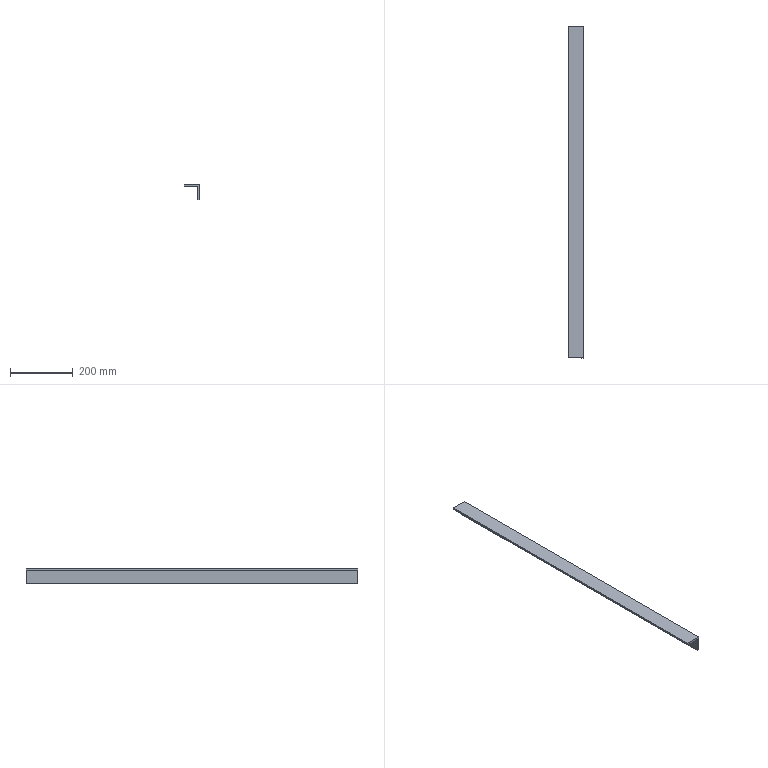Component | NX | WIDTH_CORNER_PROTECTOR | 1 solid | 8 faces | box 50 x 1054 x 50 mm | volume 594456 mm3 | plane 8
STEP:
#1=CARTESIAN_POINT('',(0.,0.,0.));
#2=DIRECTION('',(0.,0.,1.));
#3=DIRECTION('',(1.,0.,0.));
#4=AXIS2_PLACEMENT_3D('',#1,#2,#3);
#5=CARTESIAN_POINT('',(639.5,-527.,937.));
#6=VERTEX_POINT('',#5);
#7=CARTESIAN_POINT('',(639.5,-527.,987.));
#8=VERTEX_POINT('',#7);
#9=CARTESIAN_POINT('',(639.5,-527.,981.));
#10=DIRECTION('',(0.,0.,1.));
#11=VECTOR('',#10,1.);
#12=LINE('',#9,#11);
#13=CARTESIAN_POINT('',(628.5,-527.,0.));
#14=DIRECTION('',(-0.,-1.,0.));
#15=DIRECTION('',(1.,-0.,-0.));
#16=AXIS2_PLACEMENT_3D('',#13,#14,#15);
#17=PLANE('',#16);
#18=CARTESIAN_POINT('',(11.,981.));
#19=DIRECTION('',(-0.,1.));
#20=VECTOR('',#19,1.);
#21=LINE('',#18,#20);
#22=(GEOMETRIC_REPRESENTATION_CONTEXT(2)PARAMETRIC_REPRESENTATION_CONTEXT()REPRESENTATION_CONTEXT('',''));
#23=DEFINITIONAL_REPRESENTATION('',(#21),#22);
#24=PCURVE('',#17,#23);
#25=CARTESIAN_POINT('',(639.5,527.,981.));
#26=DIRECTION('',(-1.,0.,0.));
#27=DIRECTION('',(0.,0.,-1.));
#28=AXIS2_PLACEMENT_3D('',#25,#26,#27);
#29=PLANE('',#28);
#30=CARTESIAN_POINT('',(0.,1054.));
#31=DIRECTION('',(-1.,-0.));
#32=VECTOR('',#31,1.);
#33=LINE('',#30,#32);
#34=(GEOMETRIC_REPRESENTATION_CONTEXT(2)PARAMETRIC_REPRESENTATION_CONTEXT()REPRESENTATION_CONTEXT('',''));
#35=DEFINITIONAL_REPRESENTATION('',(#33),#34);
#36=PCURVE('',#29,#35);
#37=SURFACE_CURVE('',#12,(#24,#36),.PCURVE_S1.);
#38=EDGE_CURVE('',#6,#8,#37,.T.);
#39=ORIENTED_EDGE('',*,*,#38,.T.);
#40=CARTESIAN_POINT('',(589.5,-527.,987.));
#41=VERTEX_POINT('',#40);
#42=CARTESIAN_POINT('',(-628.5,-527.,987.));
#43=DIRECTION('',(-1.,0.,0.));
#44=VECTOR('',#43,1.);
#45=LINE('',#42,#44);
#46=CARTESIAN_POINT('',(-1257.,987.));
#47=DIRECTION('',(-1.,-0.));
#48=VECTOR('',#47,1.);
#49=LINE('',#46,#48);
#50=(GEOMETRIC_REPRESENTATION_CONTEXT(2)PARAMETRIC_REPRESENTATION_CONTEXT()REPRESENTATION_CONTEXT('',''));
#51=DEFINITIONAL_REPRESENTATION('',(#49),#50);
#52=PCURVE('',#17,#51);
#53=CARTESIAN_POINT('',(-628.5,527.,987.));
#54=DIRECTION('',(0.,0.,-1.));
#55=DIRECTION('',(1.,0.,0.));
#56=AXIS2_PLACEMENT_3D('',#53,#54,#55);
#57=PLANE('',#56);
#58=CARTESIAN_POINT('',(0.,1054.));
#59=DIRECTION('',(-1.,-0.));
#60=VECTOR('',#59,1.);
#61=LINE('',#58,#60);
#62=(GEOMETRIC_REPRESENTATION_CONTEXT(2)PARAMETRIC_REPRESENTATION_CONTEXT()REPRESENTATION_CONTEXT('',''));
#63=DEFINITIONAL_REPRESENTATION('',(#61),#62);
#64=PCURVE('',#57,#63);
#65=SURFACE_CURVE('',#45,(#52,#64),.PCURVE_S1.);
#66=EDGE_CURVE('',#8,#41,#65,.T.);
#67=ORIENTED_EDGE('',*,*,#66,.T.);
#68=CARTESIAN_POINT('',(589.5,-527.,981.));
#69=VERTEX_POINT('',#68);
#70=CARTESIAN_POINT('',(589.5,-527.,981.));
#71=DIRECTION('',(0.,-0.,-1.));
#72=VECTOR('',#71,1.);
#73=LINE('',#70,#72);
#74=CARTESIAN_POINT('',(-39.,981.));
#75=DIRECTION('',(0.,-1.));
#76=VECTOR('',#75,1.);
#77=LINE('',#74,#76);
#78=(GEOMETRIC_REPRESENTATION_CONTEXT(2)PARAMETRIC_REPRESENTATION_CONTEXT()REPRESENTATION_CONTEXT('',''));
#79=DEFINITIONAL_REPRESENTATION('',(#77),#78);
#80=PCURVE('',#17,#79);
#81=CARTESIAN_POINT('',(589.5,527.,981.));
#82=DIRECTION('',(1.,0.,0.));
#83=DIRECTION('',(0.,-1.,0.));
#84=AXIS2_PLACEMENT_3D('',#81,#82,#83);
#85=PLANE('',#84);
#86=CARTESIAN_POINT('',(1054.,0.));
#87=DIRECTION('',(0.,1.));
#88=VECTOR('',#87,1.);
#89=LINE('',#86,#88);
#90=(GEOMETRIC_REPRESENTATION_CONTEXT(2)PARAMETRIC_REPRESENTATION_CONTEXT()REPRESENTATION_CONTEXT('',''));
#91=DEFINITIONAL_REPRESENTATION('',(#89),#90);
#92=PCURVE('',#85,#91);
#93=SURFACE_CURVE('',#73,(#80,#92),.PCURVE_S1.);
#94=EDGE_CURVE('',#41,#69,#93,.T.);
#95=ORIENTED_EDGE('',*,*,#94,.T.);
#96=CARTESIAN_POINT('',(633.5,-527.,981.));
#97=VERTEX_POINT('',#96);
#98=CARTESIAN_POINT('',(-628.5,-527.,981.));
#99=DIRECTION('',(-1.,0.,0.));
#100=VECTOR('',#99,1.);
#101=LINE('',#98,#100);
#102=CARTESIAN_POINT('',(-1257.,981.));
#103=DIRECTION('',(-1.,-0.));
#104=VECTOR('',#103,1.);
#105=LINE('',#102,#104);
#106=(GEOMETRIC_REPRESENTATION_CONTEXT(2)PARAMETRIC_REPRESENTATION_CONTEXT()REPRESENTATION_CONTEXT('',''));
#107=DEFINITIONAL_REPRESENTATION('',(#105),#106);
#108=PCURVE('',#17,#107);
#109=CARTESIAN_POINT('',(-628.5,527.,981.));
#110=DIRECTION('',(0.,0.,-1.));
#111=DIRECTION('',(1.,0.,0.));
#112=AXIS2_PLACEMENT_3D('',#109,#110,#111);
#113=PLANE('',#112);
#114=CARTESIAN_POINT('',(0.,1054.));
#115=DIRECTION('',(-1.,-0.));
#116=VECTOR('',#115,1.);
#117=LINE('',#114,#116);
#118=(GEOMETRIC_REPRESENTATION_CONTEXT(2)PARAMETRIC_REPRESENTATION_CONTEXT()REPRESENTATION_CONTEXT('',''));
#119=DEFINITIONAL_REPRESENTATION('',(#117),#118);
#120=PCURVE('',#113,#119);
#121=SURFACE_CURVE('',#101,(#108,#120),.PCURVE_S1.);
#122=EDGE_CURVE('',#97,#69,#121,.T.);
#123=ORIENTED_EDGE('',*,*,#122,.F.);
#124=CARTESIAN_POINT('',(633.5,-527.,937.));
#125=VERTEX_POINT('',#124);
#126=CARTESIAN_POINT('',(633.5,-527.,981.));
#127=DIRECTION('',(0.,0.,1.));
#128=VECTOR('',#127,1.);
#129=LINE('',#126,#128);
#130=CARTESIAN_POINT('',(5.,981.));
#131=DIRECTION('',(-0.,1.));
#132=VECTOR('',#131,1.);
#133=LINE('',#130,#132);
#134=(GEOMETRIC_REPRESENTATION_CONTEXT(2)PARAMETRIC_REPRESENTATION_CONTEXT()REPRESENTATION_CONTEXT('',''));
#135=DEFINITIONAL_REPRESENTATION('',(#133),#134);
#136=PCURVE('',#17,#135);
#137=CARTESIAN_POINT('',(633.5,527.,981.));
#138=DIRECTION('',(-1.,0.,0.));
#139=DIRECTION('',(0.,0.,-1.));
#140=AXIS2_PLACEMENT_3D('',#137,#138,#139);
#141=PLANE('',#140);
#142=CARTESIAN_POINT('',(0.,1054.));
#143=DIRECTION('',(-1.,-0.));
#144=VECTOR('',#143,1.);
#145=LINE('',#142,#144);
#146=(GEOMETRIC_REPRESENTATION_CONTEXT(2)PARAMETRIC_REPRESENTATION_CONTEXT()REPRESENTATION_CONTEXT('',''));
#147=DEFINITIONAL_REPRESENTATION('',(#145),#146);
#148=PCURVE('',#141,#147);
#149=SURFACE_CURVE('',#129,(#136,#148),.PCURVE_S1.);
#150=EDGE_CURVE('',#125,#97,#149,.T.);
#151=ORIENTED_EDGE('',*,*,#150,.F.);
#152=CARTESIAN_POINT('',(633.5,-527.,937.));
#153=DIRECTION('',(1.,-0.,0.));
#154=VECTOR('',#153,1.);
#155=LINE('',#152,#154);
#156=CARTESIAN_POINT('',(5.,937.));
#157=DIRECTION('',(1.,0.));
#158=VECTOR('',#157,1.);
#159=LINE('',#156,#158);
#160=(GEOMETRIC_REPRESENTATION_CONTEXT(2)PARAMETRIC_REPRESENTATION_CONTEXT()REPRESENTATION_CONTEXT('',''));
#161=DEFINITIONAL_REPRESENTATION('',(#159),#160);
#162=PCURVE('',#17,#161);
#163=CARTESIAN_POINT('',(633.5,527.,937.));
#164=DIRECTION('',(0.,0.,-1.));
#165=DIRECTION('',(0.,-1.,0.));
#166=AXIS2_PLACEMENT_3D('',#163,#164,#165);
#167=PLANE('',#166);
#168=CARTESIAN_POINT('',(1054.,0.));
#169=DIRECTION('',(0.,-1.));
#170=VECTOR('',#169,1.);
#171=LINE('',#168,#170);
#172=(GEOMETRIC_REPRESENTATION_CONTEXT(2)PARAMETRIC_REPRESENTATION_CONTEXT()REPRESENTATION_CONTEXT('',''));
#173=DEFINITIONAL_REPRESENTATION('',(#171),#172);
#174=PCURVE('',#167,#173);
#175=SURFACE_CURVE('',#155,(#162,#174),.PCURVE_S1.);
#176=EDGE_CURVE('',#125,#6,#175,.T.);
#177=ORIENTED_EDGE('',*,*,#176,.T.);
#178=EDGE_LOOP('',(#39,#67,#95,#123,#151,#177));
#179=FACE_BOUND('',#178,.T.);
#180=ADVANCED_FACE('',(#179),#17,.T.);
#181=ORIENTED_EDGE('',*,*,#66,.F.);
#182=CARTESIAN_POINT('',(639.5,527.,987.));
#183=VERTEX_POINT('',#182);
#184=CARTESIAN_POINT('',(639.5,527.,987.));
#185=DIRECTION('',(0.,-1.,0.));
#186=VECTOR('',#185,1.);
#187=LINE('',#184,#186);
#188=CARTESIAN_POINT('',(1268.,0.));
#189=DIRECTION('',(0.,1.));
#190=VECTOR('',#189,1.);
#191=LINE('',#188,#190);
#192=(GEOMETRIC_REPRESENTATION_CONTEXT(2)PARAMETRIC_REPRESENTATION_CONTEXT()REPRESENTATION_CONTEXT('',''));
#193=DEFINITIONAL_REPRESENTATION('',(#191),#192);
#194=PCURVE('',#57,#193);
#195=CARTESIAN_POINT('',(-6.,0.));
#196=DIRECTION('',(0.,1.));
#197=VECTOR('',#196,1.);
#198=LINE('',#195,#197);
#199=(GEOMETRIC_REPRESENTATION_CONTEXT(2)PARAMETRIC_REPRESENTATION_CONTEXT()REPRESENTATION_CONTEXT('',''));
#200=DEFINITIONAL_REPRESENTATION('',(#198),#199);
#201=PCURVE('',#29,#200);
#202=SURFACE_CURVE('',#187,(#194,#201),.PCURVE_S1.);
#203=EDGE_CURVE('',#183,#8,#202,.T.);
#204=ORIENTED_EDGE('',*,*,#203,.F.);
#205=CARTESIAN_POINT('',(589.5,527.,987.));
#206=VERTEX_POINT('',#205);
#207=CARTESIAN_POINT('',(-628.5,527.,987.));
#208=DIRECTION('',(1.,0.,0.));
#209=VECTOR('',#208,1.);
#210=LINE('',#207,#209);
#211=CARTESIAN_POINT('',(0.,0.));
#212=DIRECTION('',(1.,0.));
#213=VECTOR('',#212,1.);
#214=LINE('',#211,#213);
#215=(GEOMETRIC_REPRESENTATION_CONTEXT(2)PARAMETRIC_REPRESENTATION_CONTEXT()REPRESENTATION_CONTEXT('',''));
#216=DEFINITIONAL_REPRESENTATION('',(#214),#215);
#217=PCURVE('',#57,#216);
#218=CARTESIAN_POINT('',(633.5,527.,981.));
#219=DIRECTION('',(0.,1.,0.));
#220=DIRECTION('',(0.,0.,-1.));
#221=AXIS2_PLACEMENT_3D('',#218,#219,#220);
#222=PLANE('',#221);
#223=CARTESIAN_POINT('',(-6.,1262.));
#224=DIRECTION('',(0.,-1.));
#225=VECTOR('',#224,1.);
#226=LINE('',#223,#225);
#227=(GEOMETRIC_REPRESENTATION_CONTEXT(2)PARAMETRIC_REPRESENTATION_CONTEXT()REPRESENTATION_CONTEXT('',''));
#228=DEFINITIONAL_REPRESENTATION('',(#226),#227);
#229=PCURVE('',#222,#228);
#230=SURFACE_CURVE('',#210,(#217,#229),.PCURVE_S1.);
#231=EDGE_CURVE('',#206,#183,#230,.T.);
#232=ORIENTED_EDGE('',*,*,#231,.F.);
#233=CARTESIAN_POINT('',(589.5,527.,987.));
#234=DIRECTION('',(0.,-1.,0.));
#235=VECTOR('',#234,1.);
#236=LINE('',#233,#235);
#237=CARTESIAN_POINT('',(1218.,0.));
#238=DIRECTION('',(0.,1.));
#239=VECTOR('',#238,1.);
#240=LINE('',#237,#239);
#241=(GEOMETRIC_REPRESENTATION_CONTEXT(2)PARAMETRIC_REPRESENTATION_CONTEXT()REPRESENTATION_CONTEXT('',''));
#242=DEFINITIONAL_REPRESENTATION('',(#240),#241);
#243=PCURVE('',#57,#242);
#244=CARTESIAN_POINT('',(0.,-6.));
#245=DIRECTION('',(1.,0.));
#246=VECTOR('',#245,1.);
#247=LINE('',#244,#246);
#248=(GEOMETRIC_REPRESENTATION_CONTEXT(2)PARAMETRIC_REPRESENTATION_CONTEXT()REPRESENTATION_CONTEXT('',''));
#249=DEFINITIONAL_REPRESENTATION('',(#247),#248);
#250=PCURVE('',#85,#249);
#251=SURFACE_CURVE('',#236,(#243,#250),.PCURVE_S1.);
#252=EDGE_CURVE('',#206,#41,#251,.T.);
#253=ORIENTED_EDGE('',*,*,#252,.T.);
#254=EDGE_LOOP('',(#181,#204,#232,#253));
#255=FACE_BOUND('',#254,.T.);
#256=ADVANCED_FACE('',(#255),#57,.F.);
#257=ORIENTED_EDGE('',*,*,#94,.F.);
#258=ORIENTED_EDGE('',*,*,#252,.F.);
#259=CARTESIAN_POINT('',(589.5,527.,981.));
#260=VERTEX_POINT('',#259);
#261=CARTESIAN_POINT('',(589.5,527.,981.));
#262=DIRECTION('',(0.,0.,1.));
#263=VECTOR('',#262,1.);
#264=LINE('',#261,#263);
#265=CARTESIAN_POINT('',(0.,0.));
#266=DIRECTION('',(0.,-1.));
#267=VECTOR('',#266,1.);
#268=LINE('',#265,#267);
#269=(GEOMETRIC_REPRESENTATION_CONTEXT(2)PARAMETRIC_REPRESENTATION_CONTEXT()REPRESENTATION_CONTEXT('',''));
#270=DEFINITIONAL_REPRESENTATION('',(#268),#269);
#271=PCURVE('',#85,#270);
#272=CARTESIAN_POINT('',(0.,44.));
#273=DIRECTION('',(-1.,0.));
#274=VECTOR('',#273,1.);
#275=LINE('',#272,#274);
#276=(GEOMETRIC_REPRESENTATION_CONTEXT(2)PARAMETRIC_REPRESENTATION_CONTEXT()REPRESENTATION_CONTEXT('',''));
#277=DEFINITIONAL_REPRESENTATION('',(#275),#276);
#278=PCURVE('',#222,#277);
#279=SURFACE_CURVE('',#264,(#271,#278),.PCURVE_S1.);
#280=EDGE_CURVE('',#260,#206,#279,.T.);
#281=ORIENTED_EDGE('',*,*,#280,.F.);
#282=CARTESIAN_POINT('',(589.5,527.,981.));
#283=DIRECTION('',(0.,-1.,0.));
#284=VECTOR('',#283,1.);
#285=LINE('',#282,#284);
#286=CARTESIAN_POINT('',(0.,0.));
#287=DIRECTION('',(1.,0.));
#288=VECTOR('',#287,1.);
#289=LINE('',#286,#288);
#290=(GEOMETRIC_REPRESENTATION_CONTEXT(2)PARAMETRIC_REPRESENTATION_CONTEXT()REPRESENTATION_CONTEXT('',''));
#291=DEFINITIONAL_REPRESENTATION('',(#289),#290);
#292=PCURVE('',#85,#291);
#293=CARTESIAN_POINT('',(1218.,0.));
#294=DIRECTION('',(0.,1.));
#295=VECTOR('',#294,1.);
#296=LINE('',#293,#295);
#297=(GEOMETRIC_REPRESENTATION_CONTEXT(2)PARAMETRIC_REPRESENTATION_CONTEXT()REPRESENTATION_CONTEXT('',''));
#298=DEFINITIONAL_REPRESENTATION('',(#296),#297);
#299=PCURVE('',#113,#298);
#300=SURFACE_CURVE('',#285,(#292,#299),.PCURVE_S1.);
#301=EDGE_CURVE('',#260,#69,#300,.T.);
#302=ORIENTED_EDGE('',*,*,#301,.T.);
#303=EDGE_LOOP('',(#257,#258,#281,#302));
#304=FACE_BOUND('',#303,.T.);
#305=ADVANCED_FACE('',(#304),#85,.F.);
#306=CARTESIAN_POINT('',(633.5,527.,981.));
#307=VERTEX_POINT('',#306);
#308=CARTESIAN_POINT('',(633.5,527.,937.));
#309=VERTEX_POINT('',#308);
#310=CARTESIAN_POINT('',(633.5,527.,981.));
#311=DIRECTION('',(0.,0.,-1.));
#312=VECTOR('',#311,1.);
#313=LINE('',#310,#312);
#314=CARTESIAN_POINT('',(0.,0.));
#315=DIRECTION('',(1.,0.));
#316=VECTOR('',#315,1.);
#317=LINE('',#314,#316);
#318=(GEOMETRIC_REPRESENTATION_CONTEXT(2)PARAMETRIC_REPRESENTATION_CONTEXT()REPRESENTATION_CONTEXT('',''));
#319=DEFINITIONAL_REPRESENTATION('',(#317),#318);
#320=PCURVE('',#222,#319);
#321=CARTESIAN_POINT('',(0.,0.));
#322=DIRECTION('',(1.,0.));
#323=VECTOR('',#322,1.);
#324=LINE('',#321,#323);
#325=(GEOMETRIC_REPRESENTATION_CONTEXT(2)PARAMETRIC_REPRESENTATION_CONTEXT()REPRESENTATION_CONTEXT('',''));
#326=DEFINITIONAL_REPRESENTATION('',(#324),#325);
#327=PCURVE('',#141,#326);
#328=SURFACE_CURVE('',#313,(#320,#327),.PCURVE_S1.);
#329=EDGE_CURVE('',#307,#309,#328,.T.);
#330=ORIENTED_EDGE('',*,*,#329,.F.);
#331=CARTESIAN_POINT('',(-628.5,527.,981.));
#332=DIRECTION('',(1.,-0.,0.));
#333=VECTOR('',#332,1.);
#334=LINE('',#331,#333);
#335=CARTESIAN_POINT('',(0.,1262.));
#336=DIRECTION('',(0.,-1.));
#337=VECTOR('',#336,1.);
#338=LINE('',#335,#337);
#339=(GEOMETRIC_REPRESENTATION_CONTEXT(2)PARAMETRIC_REPRESENTATION_CONTEXT()REPRESENTATION_CONTEXT('',''));
#340=DEFINITIONAL_REPRESENTATION('',(#338),#339);
#341=PCURVE('',#222,#340);
#342=CARTESIAN_POINT('',(0.,0.));
#343=DIRECTION('',(1.,0.));
#344=VECTOR('',#343,1.);
#345=LINE('',#342,#344);
#346=(GEOMETRIC_REPRESENTATION_CONTEXT(2)PARAMETRIC_REPRESENTATION_CONTEXT()REPRESENTATION_CONTEXT('',''));
#347=DEFINITIONAL_REPRESENTATION('',(#345),#346);
#348=PCURVE('',#113,#347);
#349=SURFACE_CURVE('',#334,(#341,#348),.PCURVE_S1.);
#350=EDGE_CURVE('',#260,#307,#349,.T.);
#351=ORIENTED_EDGE('',*,*,#350,.F.);
#352=ORIENTED_EDGE('',*,*,#280,.T.);
#353=ORIENTED_EDGE('',*,*,#231,.T.);
#354=CARTESIAN_POINT('',(639.5,527.,937.));
#355=VERTEX_POINT('',#354);
#356=CARTESIAN_POINT('',(639.5,527.,981.));
#357=DIRECTION('',(0.,0.,-1.));
#358=VECTOR('',#357,1.);
#359=LINE('',#356,#358);
#360=CARTESIAN_POINT('',(0.,-6.));
#361=DIRECTION('',(1.,0.));
#362=VECTOR('',#361,1.);
#363=LINE('',#360,#362);
#364=(GEOMETRIC_REPRESENTATION_CONTEXT(2)PARAMETRIC_REPRESENTATION_CONTEXT()REPRESENTATION_CONTEXT('',''));
#365=DEFINITIONAL_REPRESENTATION('',(#363),#364);
#366=PCURVE('',#222,#365);
#367=CARTESIAN_POINT('',(0.,0.));
#368=DIRECTION('',(1.,0.));
#369=VECTOR('',#368,1.);
#370=LINE('',#367,#369);
#371=(GEOMETRIC_REPRESENTATION_CONTEXT(2)PARAMETRIC_REPRESENTATION_CONTEXT()REPRESENTATION_CONTEXT('',''));
#372=DEFINITIONAL_REPRESENTATION('',(#370),#371);
#373=PCURVE('',#29,#372);
#374=SURFACE_CURVE('',#359,(#366,#373),.PCURVE_S1.);
#375=EDGE_CURVE('',#183,#355,#374,.T.);
#376=ORIENTED_EDGE('',*,*,#375,.T.);
#377=CARTESIAN_POINT('',(633.5,527.,937.));
#378=DIRECTION('',(1.,0.,0.));
#379=VECTOR('',#378,1.);
#380=LINE('',#377,#379);
#381=CARTESIAN_POINT('',(44.,0.));
#382=DIRECTION('',(0.,-1.));
#383=VECTOR('',#382,1.);
#384=LINE('',#381,#383);
#385=(GEOMETRIC_REPRESENTATION_CONTEXT(2)PARAMETRIC_REPRESENTATION_CONTEXT()REPRESENTATION_CONTEXT('',''));
#386=DEFINITIONAL_REPRESENTATION('',(#384),#385);
#387=PCURVE('',#222,#386);
#388=CARTESIAN_POINT('',(0.,0.));
#389=DIRECTION('',(0.,-1.));
#390=VECTOR('',#389,1.);
#391=LINE('',#388,#390);
#392=(GEOMETRIC_REPRESENTATION_CONTEXT(2)PARAMETRIC_REPRESENTATION_CONTEXT()REPRESENTATION_CONTEXT('',''));
#393=DEFINITIONAL_REPRESENTATION('',(#391),#392);
#394=PCURVE('',#167,#393);
#395=SURFACE_CURVE('',#380,(#387,#394),.PCURVE_S1.);
#396=EDGE_CURVE('',#309,#355,#395,.T.);
#397=ORIENTED_EDGE('',*,*,#396,.F.);
#398=EDGE_LOOP('',(#330,#351,#352,#353,#376,#397));
#399=FACE_BOUND('',#398,.T.);
#400=ADVANCED_FACE('',(#399),#222,.T.);
#401=CARTESIAN_POINT('',(633.5,527.,981.));
#402=DIRECTION('',(0.,-1.,0.));
#403=VECTOR('',#402,1.);
#404=LINE('',#401,#403);
#405=CARTESIAN_POINT('',(1262.,0.));
#406=DIRECTION('',(0.,1.));
#407=VECTOR('',#406,1.);
#408=LINE('',#405,#407);
#409=(GEOMETRIC_REPRESENTATION_CONTEXT(2)PARAMETRIC_REPRESENTATION_CONTEXT()REPRESENTATION_CONTEXT('',''));
#410=DEFINITIONAL_REPRESENTATION('',(#408),#409);
#411=PCURVE('',#113,#410);
#412=CARTESIAN_POINT('',(0.,0.));
#413=DIRECTION('',(0.,1.));
#414=VECTOR('',#413,1.);
#415=LINE('',#412,#414);
#416=(GEOMETRIC_REPRESENTATION_CONTEXT(2)PARAMETRIC_REPRESENTATION_CONTEXT()REPRESENTATION_CONTEXT('',''));
#417=DEFINITIONAL_REPRESENTATION('',(#415),#416);
#418=PCURVE('',#141,#417);
#419=SURFACE_CURVE('',#404,(#411,#418),.PCURVE_S1.);
#420=EDGE_CURVE('',#307,#97,#419,.T.);
#421=ORIENTED_EDGE('',*,*,#420,.T.);
#422=ORIENTED_EDGE('',*,*,#122,.T.);
#423=ORIENTED_EDGE('',*,*,#301,.F.);
#424=ORIENTED_EDGE('',*,*,#350,.T.);
#425=EDGE_LOOP('',(#421,#422,#423,#424));
#426=FACE_BOUND('',#425,.T.);
#427=ADVANCED_FACE('',(#426),#113,.T.);
#428=ORIENTED_EDGE('',*,*,#176,.F.);
#429=CARTESIAN_POINT('',(633.5,527.,937.));
#430=DIRECTION('',(0.,-1.,0.));
#431=VECTOR('',#430,1.);
#432=LINE('',#429,#431);
#433=CARTESIAN_POINT('',(0.,0.));
#434=DIRECTION('',(1.,0.));
#435=VECTOR('',#434,1.);
#436=LINE('',#433,#435);
#437=(GEOMETRIC_REPRESENTATION_CONTEXT(2)PARAMETRIC_REPRESENTATION_CONTEXT()REPRESENTATION_CONTEXT('',''));
#438=DEFINITIONAL_REPRESENTATION('',(#436),#437);
#439=PCURVE('',#167,#438);
#440=CARTESIAN_POINT('',(44.,0.));
#441=DIRECTION('',(0.,1.));
#442=VECTOR('',#441,1.);
#443=LINE('',#440,#442);
#444=(GEOMETRIC_REPRESENTATION_CONTEXT(2)PARAMETRIC_REPRESENTATION_CONTEXT()REPRESENTATION_CONTEXT('',''));
#445=DEFINITIONAL_REPRESENTATION('',(#443),#444);
#446=PCURVE('',#141,#445);
#447=SURFACE_CURVE('',#432,(#439,#446),.PCURVE_S1.);
#448=EDGE_CURVE('',#309,#125,#447,.T.);
#449=ORIENTED_EDGE('',*,*,#448,.F.);
#450=ORIENTED_EDGE('',*,*,#396,.T.);
#451=CARTESIAN_POINT('',(639.5,527.,937.));
#452=DIRECTION('',(0.,-1.,0.));
#453=VECTOR('',#452,1.);
#454=LINE('',#451,#453);
#455=CARTESIAN_POINT('',(0.,-6.));
#456=DIRECTION('',(1.,0.));
#457=VECTOR('',#456,1.);
#458=LINE('',#455,#457);
#459=(GEOMETRIC_REPRESENTATION_CONTEXT(2)PARAMETRIC_REPRESENTATION_CONTEXT()REPRESENTATION_CONTEXT('',''));
#460=DEFINITIONAL_REPRESENTATION('',(#458),#459);
#461=PCURVE('',#167,#460);
#462=CARTESIAN_POINT('',(44.,0.));
#463=DIRECTION('',(0.,1.));
#464=VECTOR('',#463,1.);
#465=LINE('',#462,#464);
#466=(GEOMETRIC_REPRESENTATION_CONTEXT(2)PARAMETRIC_REPRESENTATION_CONTEXT()REPRESENTATION_CONTEXT('',''));
#467=DEFINITIONAL_REPRESENTATION('',(#465),#466);
#468=PCURVE('',#29,#467);
#469=SURFACE_CURVE('',#454,(#461,#468),.PCURVE_S1.);
#470=EDGE_CURVE('',#355,#6,#469,.T.);
#471=ORIENTED_EDGE('',*,*,#470,.T.);
#472=EDGE_LOOP('',(#428,#449,#450,#471));
#473=FACE_BOUND('',#472,.T.);
#474=ADVANCED_FACE('',(#473),#167,.T.);
#475=ORIENTED_EDGE('',*,*,#448,.T.);
#476=ORIENTED_EDGE('',*,*,#150,.T.);
#477=ORIENTED_EDGE('',*,*,#420,.F.);
#478=ORIENTED_EDGE('',*,*,#329,.T.);
#479=EDGE_LOOP('',(#475,#476,#477,#478));
#480=FACE_BOUND('',#479,.T.);
#481=ADVANCED_FACE('',(#480),#141,.T.);
#482=ORIENTED_EDGE('',*,*,#38,.F.);
#483=ORIENTED_EDGE('',*,*,#470,.F.);
#484=ORIENTED_EDGE('',*,*,#375,.F.);
#485=ORIENTED_EDGE('',*,*,#203,.T.);
#486=EDGE_LOOP('',(#482,#483,#484,#485));
#487=FACE_BOUND('',#486,.T.);
#488=ADVANCED_FACE('',(#487),#29,.F.);
#489=CLOSED_SHELL('',(#180,#256,#305,#400,#427,#474,#481,#488));
#490=MANIFOLD_SOLID_BREP('',#489);
#491=(LENGTH_UNIT()NAMED_UNIT(*)SI_UNIT(.MILLI.,.METRE.));
#492=UNCERTAINTY_MEASURE_WITH_UNIT(LENGTH_MEASURE(0.0000001),#491,'','');
#493=(NAMED_UNIT(*)PLANE_ANGLE_UNIT()SI_UNIT($,.RADIAN.));
#494=(NAMED_UNIT(*)SI_UNIT($,.STERADIAN.)SOLID_ANGLE_UNIT());
#495=(GEOMETRIC_REPRESENTATION_CONTEXT(3)GLOBAL_UNCERTAINTY_ASSIGNED_CONTEXT((#492))GLOBAL_UNIT_ASSIGNED_CONTEXT((#491,#493,#494))REPRESENTATION_CONTEXT('',''));
#496=ADVANCED_BREP_SHAPE_REPRESENTATION('',(#4,#490),#495);